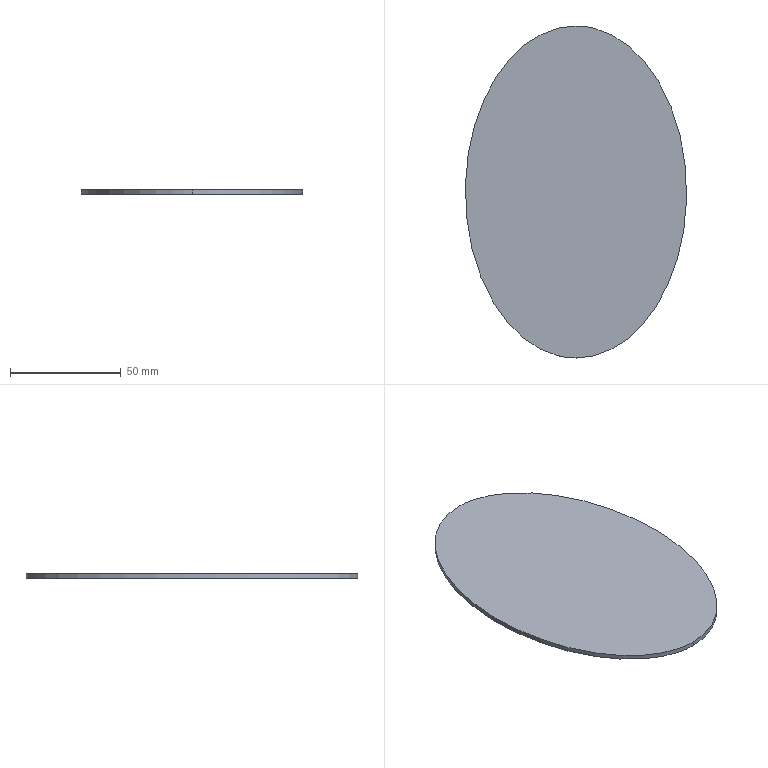Component | SolidWorks | BA850-01-03-01New-1 | 1 solid | 4 faces | box 100 x 150 x 2 mm | volume 23563 mm3 | spline 2 | plane 2 | material AISI 304
build123d program:
from build123d import *

# Parameters (mm, degrees)
SKETCH1_RX          = 75
SKETCH1_RY          = 50
BOSS_EXTRUDE1_DEPTH = 2


with BuildPart() as part:
    # Sketch1 → Boss-Extrude1 (new body)
    with BuildSketch(Plane(origin=(0, 0, 0), x_dir=(1, 0, 0), z_dir=(0, 1, 0))):
        with Locations(Location((0, 0), (0, 0, 90))):
            Ellipse(SKETCH1_RX, SKETCH1_RY)
    extrude(amount=BOSS_EXTRUDE1_DEPTH)


solid = part.part

# Placed as in the assembly
solid = solid.moved(Location((1240.186, 1138.812, 1434.454), (90, 0, 0)))
STEP:
#1=CARTESIAN_POINT('',(48.826,41.882,56.553));
#2=VERTEX_POINT('',#1);
#3=CARTESIAN_POINT('',(48.826,47.788,56.553));
#4=VERTEX_POINT('',#3);
#5=CARTESIAN_POINT('',(48.826,41.882,56.553));
#6=CARTESIAN_POINT('',(52.763,41.882,56.553));
#7=CARTESIAN_POINT('',(52.763,47.788,56.553));
#8=CARTESIAN_POINT('',(48.826,47.788,56.553));
#9=(BOUNDED_CURVE()B_SPLINE_CURVE(3,(#5,#6,#7,#8),.UNSPECIFIED.,.F.,.F.)B_SPLINE_CURVE_WITH_KNOTS((4,4),(3.142,6.283),.UNSPECIFIED.)CURVE()GEOMETRIC_REPRESENTATION_ITEM()RATIONAL_B_SPLINE_CURVE((1.,0.3333,0.3333,1.))REPRESENTATION_ITEM(''));
#10=EDGE_CURVE('',#2,#4,#9,.T.);
#11=ORIENTED_EDGE('',*,*,#10,.F.);
#12=CARTESIAN_POINT('',(48.826,41.882,56.475));
#13=VERTEX_POINT('',#12);
#14=CARTESIAN_POINT('',(48.826,41.882,56.553));
#15=DIRECTION('',(0.,0.,-1.));
#16=VECTOR('',#15,39.37);
#17=LINE('',#14,#16);
#18=EDGE_CURVE('',#2,#13,#17,.T.);
#19=ORIENTED_EDGE('',*,*,#18,.T.);
#20=CARTESIAN_POINT('',(48.826,47.788,56.475));
#21=VERTEX_POINT('',#20);
#22=CARTESIAN_POINT('',(48.826,41.882,56.475));
#23=CARTESIAN_POINT('',(52.763,41.882,56.475));
#24=CARTESIAN_POINT('',(52.763,47.788,56.475));
#25=CARTESIAN_POINT('',(48.826,47.788,56.475));
#26=(BOUNDED_CURVE()B_SPLINE_CURVE(3,(#22,#23,#24,#25),.UNSPECIFIED.,.F.,.T.)B_SPLINE_CURVE_WITH_KNOTS((4,4),(3.142,6.283),.UNSPECIFIED.)CURVE()GEOMETRIC_REPRESENTATION_ITEM()RATIONAL_B_SPLINE_CURVE((1.,0.3333,0.3333,1.))REPRESENTATION_ITEM(''));
#27=EDGE_CURVE('',#13,#21,#26,.T.);
#28=ORIENTED_EDGE('',*,*,#27,.T.);
#29=CARTESIAN_POINT('',(48.826,47.788,56.553));
#30=DIRECTION('',(0.,0.,-1.));
#31=VECTOR('',#30,39.37);
#32=LINE('',#29,#31);
#33=EDGE_CURVE('',#4,#21,#32,.T.);
#34=ORIENTED_EDGE('',*,*,#33,.F.);
#35=EDGE_LOOP('',(#11,#19,#28,#34));
#36=FACE_OUTER_BOUND('',#35,.T.);
#37=CARTESIAN_POINT('',(48.826,41.882,56.553));
#38=CARTESIAN_POINT('',(48.826,41.882,56.475));
#39=CARTESIAN_POINT('',(52.763,41.882,56.553));
#40=CARTESIAN_POINT('',(52.763,41.882,56.475));
#41=CARTESIAN_POINT('',(52.763,47.788,56.553));
#42=CARTESIAN_POINT('',(52.763,47.788,56.475));
#43=CARTESIAN_POINT('',(48.826,47.788,56.553));
#44=CARTESIAN_POINT('',(48.826,47.788,56.475));
#45=(BOUNDED_SURFACE()B_SPLINE_SURFACE(3,1,((#37,#38),(#39,#40),(#41,#42),(#43,#44)),.UNSPECIFIED.,.F.,.F.,.T.)B_SPLINE_SURFACE_WITH_KNOTS((4,4),(2,2),(0.,1.),(0.,1.),.UNSPECIFIED.)GEOMETRIC_REPRESENTATION_ITEM()RATIONAL_B_SPLINE_SURFACE(((1.,1.),(0.3333,0.3333),(0.3333,0.3333),(1.,1.)))REPRESENTATION_ITEM('')SURFACE());
#46=ADVANCED_FACE('',(#36),#45,.F.);
#47=ORIENTED_EDGE('',*,*,#18,.F.);
#48=CARTESIAN_POINT('',(48.826,47.788,56.553));
#49=CARTESIAN_POINT('',(44.889,47.788,56.553));
#50=CARTESIAN_POINT('',(44.889,41.882,56.553));
#51=CARTESIAN_POINT('',(48.826,41.882,56.553));
#52=(BOUNDED_CURVE()B_SPLINE_CURVE(3,(#48,#49,#50,#51),.UNSPECIFIED.,.F.,.F.)B_SPLINE_CURVE_WITH_KNOTS((4,4),(0.,3.142),.UNSPECIFIED.)CURVE()GEOMETRIC_REPRESENTATION_ITEM()RATIONAL_B_SPLINE_CURVE((1.,0.3333,0.3333,1.))REPRESENTATION_ITEM(''));
#53=EDGE_CURVE('',#4,#2,#52,.T.);
#54=ORIENTED_EDGE('',*,*,#53,.F.);
#55=ORIENTED_EDGE('',*,*,#33,.T.);
#56=CARTESIAN_POINT('',(48.826,47.788,56.475));
#57=CARTESIAN_POINT('',(44.889,47.788,56.475));
#58=CARTESIAN_POINT('',(44.889,41.882,56.475));
#59=CARTESIAN_POINT('',(48.826,41.882,56.475));
#60=(BOUNDED_CURVE()B_SPLINE_CURVE(3,(#56,#57,#58,#59),.UNSPECIFIED.,.F.,.F.)B_SPLINE_CURVE_WITH_KNOTS((4,4),(0.,3.142),.UNSPECIFIED.)CURVE()GEOMETRIC_REPRESENTATION_ITEM()RATIONAL_B_SPLINE_CURVE((1.,0.3333,0.3333,1.))REPRESENTATION_ITEM(''));
#61=EDGE_CURVE('',#21,#13,#60,.T.);
#62=ORIENTED_EDGE('',*,*,#61,.T.);
#63=EDGE_LOOP('',(#47,#54,#55,#62));
#64=FACE_OUTER_BOUND('',#63,.T.);
#65=CARTESIAN_POINT('',(48.826,47.788,56.553));
#66=CARTESIAN_POINT('',(48.826,47.788,56.475));
#67=CARTESIAN_POINT('',(44.889,47.788,56.553));
#68=CARTESIAN_POINT('',(44.889,47.788,56.475));
#69=CARTESIAN_POINT('',(44.889,41.882,56.553));
#70=CARTESIAN_POINT('',(44.889,41.882,56.475));
#71=CARTESIAN_POINT('',(48.826,41.882,56.553));
#72=CARTESIAN_POINT('',(48.826,41.882,56.475));
#73=(BOUNDED_SURFACE()B_SPLINE_SURFACE(3,1,((#65,#66),(#67,#68),(#69,#70),(#71,#72)),.UNSPECIFIED.,.F.,.F.,.T.)B_SPLINE_SURFACE_WITH_KNOTS((4,4),(2,2),(0.,1.),(0.,1.),.UNSPECIFIED.)GEOMETRIC_REPRESENTATION_ITEM()RATIONAL_B_SPLINE_SURFACE(((1.,1.),(0.3333,0.3333),(0.3333,0.3333),(1.,1.)))REPRESENTATION_ITEM('')SURFACE());
#74=ADVANCED_FACE('',(#64),#73,.F.);
#75=ORIENTED_EDGE('',*,*,#53,.T.);
#76=ORIENTED_EDGE('',*,*,#10,.T.);
#77=EDGE_LOOP('',(#75,#76));
#78=FACE_OUTER_BOUND('',#77,.T.);
#79=CARTESIAN_POINT('',(48.826,44.835,56.553));
#80=DIRECTION('',(0.,-0.,1.));
#81=DIRECTION('',(0.,-1.,-0.));
#82=AXIS2_PLACEMENT_3D('',#79,#80,#81);
#83=PLANE('',#82);
#84=ADVANCED_FACE('',(#78),#83,.T.);
#85=ORIENTED_EDGE('',*,*,#61,.F.);
#86=ORIENTED_EDGE('',*,*,#27,.F.);
#87=EDGE_LOOP('',(#85,#86));
#88=FACE_OUTER_BOUND('',#87,.T.);
#89=CARTESIAN_POINT('',(48.826,44.835,56.475));
#90=DIRECTION('',(0.,-0.,1.));
#91=DIRECTION('',(0.,-1.,-0.));
#92=AXIS2_PLACEMENT_3D('',#89,#90,#91);
#93=PLANE('',#92);
#94=ADVANCED_FACE('',(#88),#93,.F.);
#95=CLOSED_SHELL('',(#46,#74,#84,#94));
#96=MANIFOLD_SOLID_BREP('',#95);
#97=CARTESIAN_POINT('',(0.,0.,0.));
#98=DIRECTION('',(0.,0.,1.));
#99=DIRECTION('',(1.,0.,0.));
#100=AXIS2_PLACEMENT_3D('',#97,#98,#99);
#101=(LENGTH_UNIT()NAMED_UNIT(*)SI_UNIT($,.METRE.));
#102=LENGTH_MEASURE_WITH_UNIT(LENGTH_MEASURE(0.0254),#101);
#103=DIMENSIONAL_EXPONENTS(1.,0.,0.,0.,0.,0.,0.);
#104=(CONVERSION_BASED_UNIT('',#102)LENGTH_UNIT()NAMED_UNIT(#103));
#105=UNCERTAINTY_MEASURE_WITH_UNIT(LENGTH_MEASURE(0.00001),#104,'','');
#106=(NAMED_UNIT(*)PLANE_ANGLE_UNIT()SI_UNIT($,.RADIAN.));
#107=(NAMED_UNIT(*)SI_UNIT($,.STERADIAN.)SOLID_ANGLE_UNIT());
#108=(GEOMETRIC_REPRESENTATION_CONTEXT(3)GLOBAL_UNCERTAINTY_ASSIGNED_CONTEXT((#105))GLOBAL_UNIT_ASSIGNED_CONTEXT((#104,#106,#107))REPRESENTATION_CONTEXT('',''));
#109=ADVANCED_BREP_SHAPE_REPRESENTATION('',(#96,#100),#108);
#110=COLOUR_RGB('',0.7922,0.8196,0.9333);
#111=FILL_AREA_STYLE_COLOUR('',#110);
#112=FILL_AREA_STYLE('',(#111));
#113=SURFACE_STYLE_FILL_AREA(#112);
#114=SURFACE_SIDE_STYLE('',(#113));
#115=SURFACE_STYLE_USAGE(.BOTH.,#114);
#116=PRESENTATION_STYLE_ASSIGNMENT((#115));
#117=STYLED_ITEM('',(#116),#96);
#118=PRESENTATION_LAYER_ASSIGNMENT('','',(#117));
#119=(LENGTH_UNIT()NAMED_UNIT(*)SI_UNIT($,.METRE.));
#120=LENGTH_MEASURE_WITH_UNIT(LENGTH_MEASURE(0.0254),#119);
#121=DIMENSIONAL_EXPONENTS(1.,0.,0.,0.,0.,0.,0.);
#122=(CONVERSION_BASED_UNIT('',#120)LENGTH_UNIT()NAMED_UNIT(#121));
#123=UNCERTAINTY_MEASURE_WITH_UNIT(LENGTH_MEASURE(0.00001),#122,'','');
#124=(NAMED_UNIT(*)PLANE_ANGLE_UNIT()SI_UNIT($,.RADIAN.));
#125=(NAMED_UNIT(*)SI_UNIT($,.STERADIAN.)SOLID_ANGLE_UNIT());
#126=(GEOMETRIC_REPRESENTATION_CONTEXT(3)GLOBAL_UNCERTAINTY_ASSIGNED_CONTEXT((#123))GLOBAL_UNIT_ASSIGNED_CONTEXT((#122,#124,#125))REPRESENTATION_CONTEXT('',''));
#127=MECHANICAL_DESIGN_GEOMETRIC_PRESENTATION_REPRESENTATION('',(#117),#126);